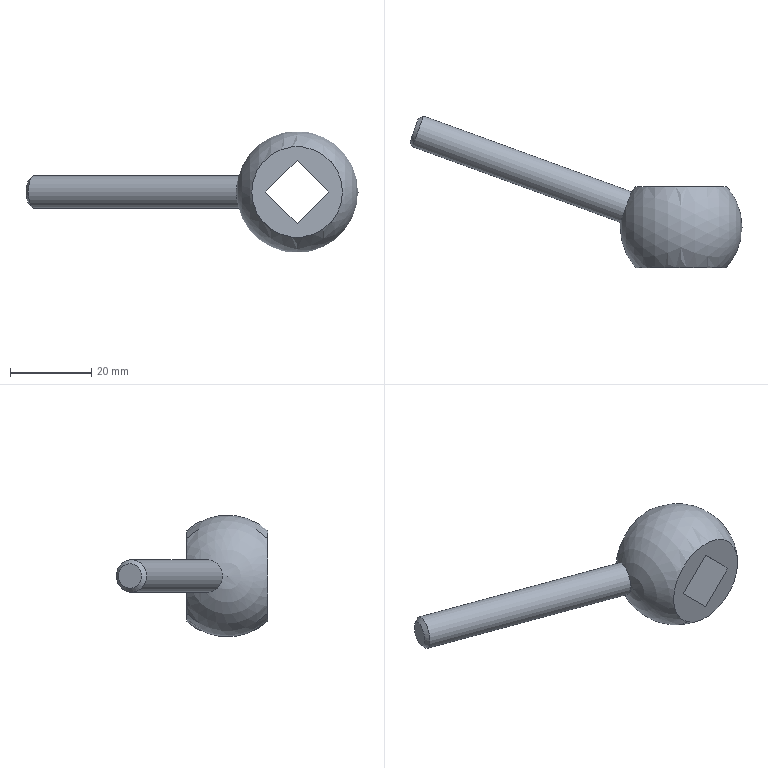Component | NX | HANDLE | 1 solid | 10 faces | box 81.8 x 37.36 x 30 mm | volume 12389 mm3 | plane 7 | sphere 1 | cylinder 1 | cone 1 | commonest cylinder face diameters 8 x1
STEP:
#1=CARTESIAN_POINT('',(0.,0.,0.));
#2=DIRECTION('',(0.,0.,1.));
#3=DIRECTION('',(1.,0.,0.));
#4=AXIS2_PLACEMENT_3D('',#1,#2,#3);
#5=CARTESIAN_POINT('',(11.18,65.,66.));
#6=VERTEX_POINT('',#5);
#7=CARTESIAN_POINT('',(0.,65.,66.));
#8=DIRECTION('',(0.,-1.,0.));
#9=DIRECTION('',(1.,0.,0.));
#10=AXIS2_PLACEMENT_3D('',#7,#8,#9);
#11=CIRCLE('',#10,11.18);
#12=CARTESIAN_POINT('',(0.,65.,66.));
#13=DIRECTION('',(0.,1.,0.));
#14=DIRECTION('',(1.,0.,0.));
#15=AXIS2_PLACEMENT_3D('',#12,#13,#14);
#16=PLANE('',#15);
#17=CARTESIAN_POINT('',(11.18,0.));
#18=CARTESIAN_POINT('',(11.18,-19.365));
#19=CARTESIAN_POINT('',(-5.59,-9.682));
#20=CARTESIAN_POINT('',(-22.361,-0.));
#21=CARTESIAN_POINT('',(-5.59,9.682));
#22=CARTESIAN_POINT('',(11.18,19.365));
#23=CARTESIAN_POINT('',(11.18,0.));
#24=(BOUNDED_CURVE()B_SPLINE_CURVE(2,(#17,#18,#19,#20,#21,#22,#23),.UNSPECIFIED.,.T.,.F.)B_SPLINE_CURVE_WITH_KNOTS((1,2,2,2,2,1),(-2.094,0.,2.094,4.189,6.283,8.378),.UNSPECIFIED.)CURVE()GEOMETRIC_REPRESENTATION_ITEM()RATIONAL_B_SPLINE_CURVE((1.,0.5,1.,0.5,1.,0.5,1.))REPRESENTATION_ITEM(''));
#25=(GEOMETRIC_REPRESENTATION_CONTEXT(2)PARAMETRIC_REPRESENTATION_CONTEXT()REPRESENTATION_CONTEXT('',''));
#26=DEFINITIONAL_REPRESENTATION('',(#24),#25);
#27=PCURVE('',#16,#26);
#28=CARTESIAN_POINT('',(0.,55.,66.));
#29=DIRECTION('',(-1.,0.,0.));
#30=DIRECTION('',(0.,1.,0.));
#31=AXIS2_PLACEMENT_3D('',#28,#29,#30);
#32=SPHERICAL_SURFACE('',#31,15.);
#33=CARTESIAN_POINT('',(6.283,-0.8411));
#34=CARTESIAN_POINT('',(6.172,-0.8417));
#35=CARTESIAN_POINT('',(5.967,-0.8094));
#36=CARTESIAN_POINT('',(5.725,-0.6857));
#37=CARTESIAN_POINT('',(5.571,-0.5142));
#38=CARTESIAN_POINT('',(5.481,-0.3169));
#39=CARTESIAN_POINT('',(5.44,-0.1069));
#40=CARTESIAN_POINT('',(5.44,0.1069));
#41=CARTESIAN_POINT('',(5.481,0.3169));
#42=CARTESIAN_POINT('',(5.571,0.5142));
#43=CARTESIAN_POINT('',(5.725,0.6856));
#44=CARTESIAN_POINT('',(5.965,0.8097));
#45=CARTESIAN_POINT('',(6.283,0.8568));
#46=CARTESIAN_POINT('',(6.601,0.8097));
#47=CARTESIAN_POINT('',(6.841,0.6856));
#48=CARTESIAN_POINT('',(6.996,0.5142));
#49=CARTESIAN_POINT('',(7.085,0.3169));
#50=CARTESIAN_POINT('',(7.126,0.1069));
#51=CARTESIAN_POINT('',(7.126,-0.1069));
#52=CARTESIAN_POINT('',(7.085,-0.3169));
#53=CARTESIAN_POINT('',(6.995,-0.5142));
#54=CARTESIAN_POINT('',(6.842,-0.6857));
#55=CARTESIAN_POINT('',(6.599,-0.8094));
#56=CARTESIAN_POINT('',(6.394,-0.8417));
#57=CARTESIAN_POINT('',(6.283,-0.8411));
#58=B_SPLINE_CURVE_WITH_KNOTS('',3,(#33,#34,#35,#36,#37,#38,#39,#40,#41,#42,#43,#44,#45,#46,#47,#48,#49,#50,#51,#52,#53,#54,#55,#56,#57),.UNSPECIFIED.,.T.,.F.,(4,1,1,1,1,1,1,1,1,1,1,1,1,1,1,1,1,1,1,1,1,1,4),(0.,0.2856,0.5712,0.8568,1.142,1.428,1.714,1.999,2.285,2.57,2.856,3.142,3.427,3.713,3.998,4.284,4.57,4.855,5.141,5.426,5.712,5.998,6.283),.QUASI_UNIFORM_KNOTS.);
#59=(GEOMETRIC_REPRESENTATION_CONTEXT(2)PARAMETRIC_REPRESENTATION_CONTEXT()REPRESENTATION_CONTEXT('',''));
#60=DEFINITIONAL_REPRESENTATION('',(#58),#59);
#61=PCURVE('',#32,#60);
#62=SURFACE_CURVE('',#11,(#27,#61),.PCURVE_S1.);
#63=EDGE_CURVE('',#6,#6,#62,.T.);
#64=ORIENTED_EDGE('',*,*,#63,.F.);
#65=EDGE_LOOP('',(#64));
#66=FACE_BOUND('',#65,.T.);
#67=CARTESIAN_POINT('',(0.,65.,58.222));
#68=VERTEX_POINT('',#67);
#69=CARTESIAN_POINT('',(7.778,65.,66.));
#70=VERTEX_POINT('',#69);
#71=CARTESIAN_POINT('',(3.889,65.,62.111));
#72=DIRECTION('',(0.7071,0.,0.7071));
#73=VECTOR('',#72,1.);
#74=LINE('',#71,#73);
#75=CARTESIAN_POINT('',(3.889,3.889));
#76=DIRECTION('',(0.7071,-0.7071));
#77=VECTOR('',#76,1.);
#78=LINE('',#75,#77);
#79=(GEOMETRIC_REPRESENTATION_CONTEXT(2)PARAMETRIC_REPRESENTATION_CONTEXT()REPRESENTATION_CONTEXT('',''));
#80=DEFINITIONAL_REPRESENTATION('',(#78),#79);
#81=PCURVE('',#16,#80);
#82=CARTESIAN_POINT('',(7.778,86.,66.));
#83=DIRECTION('',(-0.7071,0.,0.7071));
#84=DIRECTION('',(0.7071,0.,0.7071));
#85=AXIS2_PLACEMENT_3D('',#82,#83,#84);
#86=PLANE('',#85);
#87=CARTESIAN_POINT('',(-5.5,-21.));
#88=DIRECTION('',(1.,0.));
#89=VECTOR('',#88,1.);
#90=LINE('',#87,#89);
#91=(GEOMETRIC_REPRESENTATION_CONTEXT(2)PARAMETRIC_REPRESENTATION_CONTEXT()REPRESENTATION_CONTEXT('',''));
#92=DEFINITIONAL_REPRESENTATION('',(#90),#91);
#93=PCURVE('',#86,#92);
#94=SURFACE_CURVE('',#74,(#81,#93),.PCURVE_S1.);
#95=EDGE_CURVE('',#68,#70,#94,.T.);
#96=ORIENTED_EDGE('',*,*,#95,.T.);
#97=CARTESIAN_POINT('',(0.,65.,73.778));
#98=VERTEX_POINT('',#97);
#99=CARTESIAN_POINT('',(3.889,65.,69.889));
#100=DIRECTION('',(-0.7071,0.,0.7071));
#101=VECTOR('',#100,1.);
#102=LINE('',#99,#101);
#103=CARTESIAN_POINT('',(3.889,-3.889));
#104=DIRECTION('',(-0.7071,-0.7071));
#105=VECTOR('',#104,1.);
#106=LINE('',#103,#105);
#107=(GEOMETRIC_REPRESENTATION_CONTEXT(2)PARAMETRIC_REPRESENTATION_CONTEXT()REPRESENTATION_CONTEXT('',''));
#108=DEFINITIONAL_REPRESENTATION('',(#106),#107);
#109=PCURVE('',#16,#108);
#110=CARTESIAN_POINT('',(0.,86.,73.778));
#111=DIRECTION('',(-0.7071,0.,-0.7071));
#112=DIRECTION('',(-0.7071,0.,0.7071));
#113=AXIS2_PLACEMENT_3D('',#110,#111,#112);
#114=PLANE('',#113);
#115=CARTESIAN_POINT('',(-5.5,-21.));
#116=DIRECTION('',(1.,0.));
#117=VECTOR('',#116,1.);
#118=LINE('',#115,#117);
#119=(GEOMETRIC_REPRESENTATION_CONTEXT(2)PARAMETRIC_REPRESENTATION_CONTEXT()REPRESENTATION_CONTEXT('',''));
#120=DEFINITIONAL_REPRESENTATION('',(#118),#119);
#121=PCURVE('',#114,#120);
#122=SURFACE_CURVE('',#102,(#109,#121),.PCURVE_S1.);
#123=EDGE_CURVE('',#70,#98,#122,.T.);
#124=ORIENTED_EDGE('',*,*,#123,.T.);
#125=CARTESIAN_POINT('',(-7.778,65.,66.));
#126=VERTEX_POINT('',#125);
#127=CARTESIAN_POINT('',(-3.889,65.,69.889));
#128=DIRECTION('',(-0.7071,0.,-0.7071));
#129=VECTOR('',#128,1.);
#130=LINE('',#127,#129);
#131=CARTESIAN_POINT('',(-3.889,-3.889));
#132=DIRECTION('',(-0.7071,0.7071));
#133=VECTOR('',#132,1.);
#134=LINE('',#131,#133);
#135=(GEOMETRIC_REPRESENTATION_CONTEXT(2)PARAMETRIC_REPRESENTATION_CONTEXT()REPRESENTATION_CONTEXT('',''));
#136=DEFINITIONAL_REPRESENTATION('',(#134),#135);
#137=PCURVE('',#16,#136);
#138=CARTESIAN_POINT('',(-7.778,86.,66.));
#139=DIRECTION('',(0.7071,0.,-0.7071));
#140=DIRECTION('',(-0.7071,0.,-0.7071));
#141=AXIS2_PLACEMENT_3D('',#138,#139,#140);
#142=PLANE('',#141);
#143=CARTESIAN_POINT('',(-5.5,-21.));
#144=DIRECTION('',(1.,0.));
#145=VECTOR('',#144,1.);
#146=LINE('',#143,#145);
#147=(GEOMETRIC_REPRESENTATION_CONTEXT(2)PARAMETRIC_REPRESENTATION_CONTEXT()REPRESENTATION_CONTEXT('',''));
#148=DEFINITIONAL_REPRESENTATION('',(#146),#147);
#149=PCURVE('',#142,#148);
#150=SURFACE_CURVE('',#130,(#137,#149),.PCURVE_S1.);
#151=EDGE_CURVE('',#98,#126,#150,.T.);
#152=ORIENTED_EDGE('',*,*,#151,.T.);
#153=CARTESIAN_POINT('',(-3.889,65.,62.111));
#154=DIRECTION('',(0.7071,0.,-0.7071));
#155=VECTOR('',#154,1.);
#156=LINE('',#153,#155);
#157=CARTESIAN_POINT('',(-3.889,3.889));
#158=DIRECTION('',(0.7071,0.7071));
#159=VECTOR('',#158,1.);
#160=LINE('',#157,#159);
#161=(GEOMETRIC_REPRESENTATION_CONTEXT(2)PARAMETRIC_REPRESENTATION_CONTEXT()REPRESENTATION_CONTEXT('',''));
#162=DEFINITIONAL_REPRESENTATION('',(#160),#161);
#163=PCURVE('',#16,#162);
#164=CARTESIAN_POINT('',(0.,86.,58.222));
#165=DIRECTION('',(0.7071,0.,0.7071));
#166=DIRECTION('',(0.7071,0.,-0.7071));
#167=AXIS2_PLACEMENT_3D('',#164,#165,#166);
#168=PLANE('',#167);
#169=CARTESIAN_POINT('',(-5.5,-21.));
#170=DIRECTION('',(1.,0.));
#171=VECTOR('',#170,1.);
#172=LINE('',#169,#171);
#173=(GEOMETRIC_REPRESENTATION_CONTEXT(2)PARAMETRIC_REPRESENTATION_CONTEXT()REPRESENTATION_CONTEXT('',''));
#174=DEFINITIONAL_REPRESENTATION('',(#172),#173);
#175=PCURVE('',#168,#174);
#176=SURFACE_CURVE('',#156,(#163,#175),.PCURVE_S1.);
#177=EDGE_CURVE('',#126,#68,#176,.T.);
#178=ORIENTED_EDGE('',*,*,#177,.T.);
#179=EDGE_LOOP('',(#96,#124,#152,#178));
#180=FACE_BOUND('',#179,.T.);
#181=ADVANCED_FACE('',(#66,#180),#16,.T.);
#182=CARTESIAN_POINT('',(-11.18,45.,66.));
#183=VERTEX_POINT('',#182);
#184=CARTESIAN_POINT('',(0.,45.,66.));
#185=DIRECTION('',(0.,1.,0.));
#186=DIRECTION('',(-1.,0.,0.));
#187=AXIS2_PLACEMENT_3D('',#184,#185,#186);
#188=CIRCLE('',#187,11.18);
#189=CARTESIAN_POINT('',(0.,45.,66.));
#190=DIRECTION('',(0.,-1.,0.));
#191=DIRECTION('',(-1.,0.,0.));
#192=AXIS2_PLACEMENT_3D('',#189,#190,#191);
#193=PLANE('',#192);
#194=CARTESIAN_POINT('',(11.18,0.));
#195=CARTESIAN_POINT('',(11.18,-19.365));
#196=CARTESIAN_POINT('',(-5.59,-9.682));
#197=CARTESIAN_POINT('',(-22.361,-0.));
#198=CARTESIAN_POINT('',(-5.59,9.682));
#199=CARTESIAN_POINT('',(11.18,19.365));
#200=CARTESIAN_POINT('',(11.18,0.));
#201=(BOUNDED_CURVE()B_SPLINE_CURVE(2,(#194,#195,#196,#197,#198,#199,#200),.UNSPECIFIED.,.T.,.F.)B_SPLINE_CURVE_WITH_KNOTS((1,2,2,2,2,1),(-2.094,0.,2.094,4.189,6.283,8.378),.UNSPECIFIED.)CURVE()GEOMETRIC_REPRESENTATION_ITEM()RATIONAL_B_SPLINE_CURVE((1.,0.5,1.,0.5,1.,0.5,1.))REPRESENTATION_ITEM(''));
#202=(GEOMETRIC_REPRESENTATION_CONTEXT(2)PARAMETRIC_REPRESENTATION_CONTEXT()REPRESENTATION_CONTEXT('',''));
#203=DEFINITIONAL_REPRESENTATION('',(#201),#202);
#204=PCURVE('',#193,#203);
#205=CARTESIAN_POINT('',(9.425,0.8411));
#206=CARTESIAN_POINT('',(9.536,0.8417));
#207=CARTESIAN_POINT('',(9.741,0.8094));
#208=CARTESIAN_POINT('',(9.983,0.6857));
#209=CARTESIAN_POINT('',(10.137,0.5142));
#210=CARTESIAN_POINT('',(10.227,0.3169));
#211=CARTESIAN_POINT('',(10.268,0.1069));
#212=CARTESIAN_POINT('',(10.268,-0.1069));
#213=CARTESIAN_POINT('',(10.227,-0.3169));
#214=CARTESIAN_POINT('',(10.137,-0.5142));
#215=CARTESIAN_POINT('',(9.983,-0.6856));
#216=CARTESIAN_POINT('',(9.743,-0.8097));
#217=CARTESIAN_POINT('',(9.425,-0.8568));
#218=CARTESIAN_POINT('',(9.107,-0.8097));
#219=CARTESIAN_POINT('',(8.867,-0.6856));
#220=CARTESIAN_POINT('',(8.712,-0.5142));
#221=CARTESIAN_POINT('',(8.623,-0.3169));
#222=CARTESIAN_POINT('',(8.582,-0.1069));
#223=CARTESIAN_POINT('',(8.582,0.1069));
#224=CARTESIAN_POINT('',(8.623,0.3169));
#225=CARTESIAN_POINT('',(8.713,0.5142));
#226=CARTESIAN_POINT('',(8.866,0.6857));
#227=CARTESIAN_POINT('',(9.109,0.8094));
#228=CARTESIAN_POINT('',(9.314,0.8417));
#229=CARTESIAN_POINT('',(9.425,0.8411));
#230=B_SPLINE_CURVE_WITH_KNOTS('',3,(#205,#206,#207,#208,#209,#210,#211,#212,#213,#214,#215,#216,#217,#218,#219,#220,#221,#222,#223,#224,#225,#226,#227,#228,#229),.UNSPECIFIED.,.T.,.F.,(4,1,1,1,1,1,1,1,1,1,1,1,1,1,1,1,1,1,1,1,1,1,4),(0.,0.2856,0.5712,0.8568,1.142,1.428,1.714,1.999,2.285,2.57,2.856,3.142,3.427,3.713,3.998,4.284,4.57,4.855,5.141,5.426,5.712,5.998,6.283),.QUASI_UNIFORM_KNOTS.);
#231=(GEOMETRIC_REPRESENTATION_CONTEXT(2)PARAMETRIC_REPRESENTATION_CONTEXT()REPRESENTATION_CONTEXT('',''));
#232=DEFINITIONAL_REPRESENTATION('',(#230),#231);
#233=PCURVE('',#32,#232);
#234=SURFACE_CURVE('',#188,(#204,#233),.PCURVE_S1.);
#235=EDGE_CURVE('',#183,#183,#234,.T.);
#236=ORIENTED_EDGE('',*,*,#235,.F.);
#237=EDGE_LOOP('',(#236));
#238=FACE_BOUND('',#237,.T.);
#239=CARTESIAN_POINT('',(-7.778,45.,66.));
#240=VERTEX_POINT('',#239);
#241=CARTESIAN_POINT('',(0.,45.,73.778));
#242=VERTEX_POINT('',#241);
#243=CARTESIAN_POINT('',(-3.889,45.,69.889));
#244=DIRECTION('',(0.7071,0.,0.7071));
#245=VECTOR('',#244,1.);
#246=LINE('',#243,#245);
#247=CARTESIAN_POINT('',(3.889,-3.889));
#248=DIRECTION('',(-0.7071,-0.7071));
#249=VECTOR('',#248,1.);
#250=LINE('',#247,#249);
#251=(GEOMETRIC_REPRESENTATION_CONTEXT(2)PARAMETRIC_REPRESENTATION_CONTEXT()REPRESENTATION_CONTEXT('',''));
#252=DEFINITIONAL_REPRESENTATION('',(#250),#251);
#253=PCURVE('',#193,#252);
#254=CARTESIAN_POINT('',(-5.5,-41.));
#255=DIRECTION('',(-1.,0.));
#256=VECTOR('',#255,1.);
#257=LINE('',#254,#256);
#258=(GEOMETRIC_REPRESENTATION_CONTEXT(2)PARAMETRIC_REPRESENTATION_CONTEXT()REPRESENTATION_CONTEXT('',''));
#259=DEFINITIONAL_REPRESENTATION('',(#257),#258);
#260=PCURVE('',#142,#259);
#261=SURFACE_CURVE('',#246,(#253,#260),.PCURVE_S1.);
#262=EDGE_CURVE('',#240,#242,#261,.T.);
#263=ORIENTED_EDGE('',*,*,#262,.T.);
#264=CARTESIAN_POINT('',(7.778,45.,66.));
#265=VERTEX_POINT('',#264);
#266=CARTESIAN_POINT('',(3.889,45.,69.889));
#267=DIRECTION('',(0.7071,0.,-0.7071));
#268=VECTOR('',#267,1.);
#269=LINE('',#266,#268);
#270=CARTESIAN_POINT('',(-3.889,-3.889));
#271=DIRECTION('',(-0.7071,0.7071));
#272=VECTOR('',#271,1.);
#273=LINE('',#270,#272);
#274=(GEOMETRIC_REPRESENTATION_CONTEXT(2)PARAMETRIC_REPRESENTATION_CONTEXT()REPRESENTATION_CONTEXT('',''));
#275=DEFINITIONAL_REPRESENTATION('',(#273),#274);
#276=PCURVE('',#193,#275);
#277=CARTESIAN_POINT('',(-5.5,-41.));
#278=DIRECTION('',(-1.,0.));
#279=VECTOR('',#278,1.);
#280=LINE('',#277,#279);
#281=(GEOMETRIC_REPRESENTATION_CONTEXT(2)PARAMETRIC_REPRESENTATION_CONTEXT()REPRESENTATION_CONTEXT('',''));
#282=DEFINITIONAL_REPRESENTATION('',(#280),#281);
#283=PCURVE('',#114,#282);
#284=SURFACE_CURVE('',#269,(#276,#283),.PCURVE_S1.);
#285=EDGE_CURVE('',#242,#265,#284,.T.);
#286=ORIENTED_EDGE('',*,*,#285,.T.);
#287=CARTESIAN_POINT('',(0.,45.,58.222));
#288=VERTEX_POINT('',#287);
#289=CARTESIAN_POINT('',(3.889,45.,62.111));
#290=DIRECTION('',(-0.7071,0.,-0.7071));
#291=VECTOR('',#290,1.);
#292=LINE('',#289,#291);
#293=CARTESIAN_POINT('',(-3.889,3.889));
#294=DIRECTION('',(0.7071,0.7071));
#295=VECTOR('',#294,1.);
#296=LINE('',#293,#295);
#297=(GEOMETRIC_REPRESENTATION_CONTEXT(2)PARAMETRIC_REPRESENTATION_CONTEXT()REPRESENTATION_CONTEXT('',''));
#298=DEFINITIONAL_REPRESENTATION('',(#296),#297);
#299=PCURVE('',#193,#298);
#300=CARTESIAN_POINT('',(-5.5,-41.));
#301=DIRECTION('',(-1.,0.));
#302=VECTOR('',#301,1.);
#303=LINE('',#300,#302);
#304=(GEOMETRIC_REPRESENTATION_CONTEXT(2)PARAMETRIC_REPRESENTATION_CONTEXT()REPRESENTATION_CONTEXT('',''));
#305=DEFINITIONAL_REPRESENTATION('',(#303),#304);
#306=PCURVE('',#86,#305);
#307=SURFACE_CURVE('',#292,(#299,#306),.PCURVE_S1.);
#308=EDGE_CURVE('',#265,#288,#307,.T.);
#309=ORIENTED_EDGE('',*,*,#308,.T.);
#310=CARTESIAN_POINT('',(-3.889,45.,62.111));
#311=DIRECTION('',(-0.7071,0.,0.7071));
#312=VECTOR('',#311,1.);
#313=LINE('',#310,#312);
#314=CARTESIAN_POINT('',(3.889,3.889));
#315=DIRECTION('',(0.7071,-0.7071));
#316=VECTOR('',#315,1.);
#317=LINE('',#314,#316);
#318=(GEOMETRIC_REPRESENTATION_CONTEXT(2)PARAMETRIC_REPRESENTATION_CONTEXT()REPRESENTATION_CONTEXT('',''));
#319=DEFINITIONAL_REPRESENTATION('',(#317),#318);
#320=PCURVE('',#193,#319);
#321=CARTESIAN_POINT('',(-5.5,-41.));
#322=DIRECTION('',(-1.,0.));
#323=VECTOR('',#322,1.);
#324=LINE('',#321,#323);
#325=(GEOMETRIC_REPRESENTATION_CONTEXT(2)PARAMETRIC_REPRESENTATION_CONTEXT()REPRESENTATION_CONTEXT('',''));
#326=DEFINITIONAL_REPRESENTATION('',(#324),#325);
#327=PCURVE('',#168,#326);
#328=SURFACE_CURVE('',#313,(#320,#327),.PCURVE_S1.);
#329=EDGE_CURVE('',#288,#240,#328,.T.);
#330=ORIENTED_EDGE('',*,*,#329,.T.);
#331=EDGE_LOOP('',(#263,#286,#309,#330));
#332=FACE_BOUND('',#331,.T.);
#333=ADVANCED_FACE('',(#238,#332),#193,.T.);
#334=ORIENTED_EDGE('',*,*,#235,.T.);
#335=EDGE_LOOP('',(#334));
#336=FACE_BOUND('',#335,.T.);
#337=ORIENTED_EDGE('',*,*,#63,.T.);
#338=EDGE_LOOP('',(#337));
#339=FACE_BOUND('',#338,.T.);
#340=CARTESIAN_POINT('',(-14.953,56.186,66.));
#341=VERTEX_POINT('',#340);
#342=CARTESIAN_POINT('',(-13.585,59.945,66.));
#343=DIRECTION('',(0.9397,-0.342,0.));
#344=DIRECTION('',(-0.342,-0.9397,0.));
#345=AXIS2_PLACEMENT_3D('',#342,#343,#344);
#346=CIRCLE('',#345,4.);
#347=CARTESIAN_POINT('',(6.283,1.492));
#348=CARTESIAN_POINT('',(6.641,1.488));
#349=CARTESIAN_POINT('',(7.072,1.46));
#350=CARTESIAN_POINT('',(7.185,1.383));
#351=CARTESIAN_POINT('',(7.176,1.307));
#352=CARTESIAN_POINT('',(7.109,1.232));
#353=CARTESIAN_POINT('',(7.017,1.163));
#354=CARTESIAN_POINT('',(6.91,1.102));
#355=CARTESIAN_POINT('',(6.794,1.049));
#356=CARTESIAN_POINT('',(6.671,1.006));
#357=CARTESIAN_POINT('',(6.544,0.9752));
#358=CARTESIAN_POINT('',(6.414,0.9561));
#359=CARTESIAN_POINT('',(6.283,0.9497));
#360=CARTESIAN_POINT('',(6.152,0.9561));
#361=CARTESIAN_POINT('',(6.022,0.9752));
#362=CARTESIAN_POINT('',(5.895,1.006));
#363=CARTESIAN_POINT('',(5.772,1.049));
#364=CARTESIAN_POINT('',(5.656,1.102));
#365=CARTESIAN_POINT('',(5.549,1.163));
#366=CARTESIAN_POINT('',(5.457,1.232));
#367=CARTESIAN_POINT('',(5.39,1.307));
#368=CARTESIAN_POINT('',(5.382,1.383));
#369=CARTESIAN_POINT('',(5.494,1.46));
#370=CARTESIAN_POINT('',(5.926,1.488));
#371=CARTESIAN_POINT('',(6.283,1.492));
#372=B_SPLINE_CURVE_WITH_KNOTS('',3,(#347,#348,#349,#350,#351,#352,#353,#354,#355,#356,#357,#358,#359,#360,#361,#362,#363,#364,#365,#366,#367,#368,#369,#370,#371),.UNSPECIFIED.,.T.,.F.,(4,1,1,1,1,1,1,1,1,1,1,1,1,1,1,1,1,1,1,1,1,1,4),(0.,0.2856,0.5712,0.8568,1.142,1.428,1.714,1.999,2.285,2.57,2.856,3.142,3.427,3.713,3.998,4.284,4.57,4.855,5.141,5.426,5.712,5.998,6.283),.QUASI_UNIFORM_KNOTS.);
#373=(GEOMETRIC_REPRESENTATION_CONTEXT(2)PARAMETRIC_REPRESENTATION_CONTEXT()REPRESENTATION_CONTEXT('',''));
#374=DEFINITIONAL_REPRESENTATION('',(#372),#373);
#375=PCURVE('',#32,#374);
#376=CARTESIAN_POINT('',(0.,55.,66.));
#377=DIRECTION('',(-0.9397,0.342,0.));
#378=DIRECTION('',(0.342,0.9397,0.));
#379=AXIS2_PLACEMENT_3D('',#376,#377,#378);
#380=CYLINDRICAL_SURFACE('',#379,4.);
#381=CARTESIAN_POINT('',(9.425,14.457));
#382=DIRECTION('',(-1.,0.));
#383=VECTOR('',#382,1.);
#384=LINE('',#381,#383);
#385=(GEOMETRIC_REPRESENTATION_CONTEXT(2)PARAMETRIC_REPRESENTATION_CONTEXT()REPRESENTATION_CONTEXT('',''));
#386=DEFINITIONAL_REPRESENTATION('',(#384),#385);
#387=PCURVE('',#380,#386);
#388=SURFACE_CURVE('',#346,(#375,#387),.PCURVE_S1.);
#389=EDGE_CURVE('',#341,#341,#388,.T.);
#390=ORIENTED_EDGE('',*,*,#389,.T.);
#391=EDGE_LOOP('',(#390));
#392=FACE_BOUND('',#391,.T.);
#393=CARTESIAN_POINT('',(15.,55.,66.));
#394=VERTEX_POINT('',#393);
#395=VERTEX_LOOP('',#394);
#396=FACE_BOUND('',#395,.T.);
#397=ADVANCED_FACE('',(#336,#339,#392,#396),#32,.T.);
#398=CARTESIAN_POINT('',(-66.207,74.841,66.));
#399=VERTEX_POINT('',#398);
#400=CARTESIAN_POINT('',(-64.839,78.599,66.));
#401=DIRECTION('',(0.9397,-0.342,0.));
#402=DIRECTION('',(-0.342,-0.9397,0.));
#403=AXIS2_PLACEMENT_3D('',#400,#401,#402);
#404=CIRCLE('',#403,4.);
#405=CARTESIAN_POINT('',(9.425,69.));
#406=DIRECTION('',(-1.,0.));
#407=VECTOR('',#406,1.);
#408=LINE('',#405,#407);
#409=(GEOMETRIC_REPRESENTATION_CONTEXT(2)PARAMETRIC_REPRESENTATION_CONTEXT()REPRESENTATION_CONTEXT('',''));
#410=DEFINITIONAL_REPRESENTATION('',(#408),#409);
#411=PCURVE('',#380,#410);
#412=CARTESIAN_POINT('',(-64.839,78.599,66.));
#413=DIRECTION('',(0.9397,-0.342,0.));
#414=DIRECTION('',(-0.342,-0.9397,0.));
#415=AXIS2_PLACEMENT_3D('',#412,#413,#414);
#416=CONICAL_SURFACE('',#415,4.,0.7854);
#417=CARTESIAN_POINT('',(0.,0.));
#418=DIRECTION('',(1.,0.));
#419=VECTOR('',#418,1.);
#420=LINE('',#417,#419);
#421=(GEOMETRIC_REPRESENTATION_CONTEXT(2)PARAMETRIC_REPRESENTATION_CONTEXT()REPRESENTATION_CONTEXT('',''));
#422=DEFINITIONAL_REPRESENTATION('',(#420),#421);
#423=PCURVE('',#416,#422);
#424=SURFACE_CURVE('',#404,(#411,#423),.PCURVE_S1.);
#425=EDGE_CURVE('',#399,#399,#424,.T.);
#426=ORIENTED_EDGE('',*,*,#425,.T.);
#427=CARTESIAN_POINT('',(-14.953,56.186,66.));
#428=CARTESIAN_POINT('',(-66.207,74.841,66.));
#429=B_SPLINE_CURVE_WITH_KNOTS('',1,(#427,#428),.UNSPECIFIED.,.F.,.F.,(2,2),(14.457,69.),.PIECEWISE_BEZIER_KNOTS.);
#430=CARTESIAN_POINT('',(3.142,0.));
#431=DIRECTION('',(0.,1.));
#432=VECTOR('',#431,1.);
#433=LINE('',#430,#432);
#434=(GEOMETRIC_REPRESENTATION_CONTEXT(2)PARAMETRIC_REPRESENTATION_CONTEXT()REPRESENTATION_CONTEXT('',''));
#435=DEFINITIONAL_REPRESENTATION('',(#433),#434);
#436=PCURVE('',#380,#435);
#437=CARTESIAN_POINT('',(9.425,0.));
#438=DIRECTION('',(0.,1.));
#439=VECTOR('',#438,1.);
#440=LINE('',#437,#439);
#441=(GEOMETRIC_REPRESENTATION_CONTEXT(2)PARAMETRIC_REPRESENTATION_CONTEXT()REPRESENTATION_CONTEXT('',''));
#442=DEFINITIONAL_REPRESENTATION('',(#440),#441);
#443=PCURVE('',#380,#442);
#444=SEAM_CURVE('',#429,(#436,#443),.PCURVE_S1.);
#445=EDGE_CURVE('',#341,#399,#444,.T.);
#446=ORIENTED_EDGE('',*,*,#445,.F.);
#447=ORIENTED_EDGE('',*,*,#389,.F.);
#448=ORIENTED_EDGE('',*,*,#445,.T.);
#449=EDGE_LOOP('',(#426,#446,#447,#448));
#450=FACE_BOUND('',#449,.T.);
#451=ADVANCED_FACE('',(#450),#380,.T.);
#452=CARTESIAN_POINT('',(-66.805,76.122,66.));
#453=VERTEX_POINT('',#452);
#454=CARTESIAN_POINT('',(-65.778,78.941,66.));
#455=DIRECTION('',(-0.9397,0.342,0.));
#456=DIRECTION('',(-0.342,-0.9397,0.));
#457=AXIS2_PLACEMENT_3D('',#454,#455,#456);
#458=CIRCLE('',#457,3.);
#459=CARTESIAN_POINT('',(-65.778,78.941,66.));
#460=DIRECTION('',(0.9397,-0.342,0.));
#461=DIRECTION('',(-0.342,-0.9397,0.));
#462=AXIS2_PLACEMENT_3D('',#459,#460,#461);
#463=PLANE('',#462);
#464=CARTESIAN_POINT('',(3.,0.));
#465=CARTESIAN_POINT('',(3.,-5.196));
#466=CARTESIAN_POINT('',(-1.5,-2.598));
#467=CARTESIAN_POINT('',(-6.,-0.));
#468=CARTESIAN_POINT('',(-1.5,2.598));
#469=CARTESIAN_POINT('',(3.,5.196));
#470=CARTESIAN_POINT('',(3.,0.));
#471=(BOUNDED_CURVE()B_SPLINE_CURVE(2,(#464,#465,#466,#467,#468,#469,#470),.UNSPECIFIED.,.T.,.F.)B_SPLINE_CURVE_WITH_KNOTS((1,2,2,2,2,1),(-2.094,0.,2.094,4.189,6.283,8.378),.UNSPECIFIED.)CURVE()GEOMETRIC_REPRESENTATION_ITEM()RATIONAL_B_SPLINE_CURVE((1.,0.5,1.,0.5,1.,0.5,1.))REPRESENTATION_ITEM(''));
#472=(GEOMETRIC_REPRESENTATION_CONTEXT(2)PARAMETRIC_REPRESENTATION_CONTEXT()REPRESENTATION_CONTEXT('',''));
#473=DEFINITIONAL_REPRESENTATION('',(#471),#472);
#474=PCURVE('',#463,#473);
#475=CARTESIAN_POINT('',(6.283,-1.));
#476=DIRECTION('',(-1.,0.));
#477=VECTOR('',#476,1.);
#478=LINE('',#475,#477);
#479=(GEOMETRIC_REPRESENTATION_CONTEXT(2)PARAMETRIC_REPRESENTATION_CONTEXT()REPRESENTATION_CONTEXT('',''));
#480=DEFINITIONAL_REPRESENTATION('',(#478),#479);
#481=PCURVE('',#416,#480);
#482=SURFACE_CURVE('',#458,(#474,#481),.PCURVE_S1.);
#483=EDGE_CURVE('',#453,#453,#482,.T.);
#484=ORIENTED_EDGE('',*,*,#483,.T.);
#485=EDGE_LOOP('',(#484));
#486=FACE_BOUND('',#485,.T.);
#487=ADVANCED_FACE('',(#486),#463,.F.);
#488=CARTESIAN_POINT('',(7.778,86.,66.));
#489=DIRECTION('',(0.,1.,0.));
#490=VECTOR('',#489,1.);
#491=LINE('',#488,#490);
#492=CARTESIAN_POINT('',(-11.,0.));
#493=DIRECTION('',(0.,1.));
#494=VECTOR('',#493,1.);
#495=LINE('',#492,#494);
#496=(GEOMETRIC_REPRESENTATION_CONTEXT(2)PARAMETRIC_REPRESENTATION_CONTEXT()REPRESENTATION_CONTEXT('',''));
#497=DEFINITIONAL_REPRESENTATION('',(#495),#496);
#498=PCURVE('',#114,#497);
#499=CARTESIAN_POINT('',(0.,0.));
#500=DIRECTION('',(0.,1.));
#501=VECTOR('',#500,1.);
#502=LINE('',#499,#501);
#503=(GEOMETRIC_REPRESENTATION_CONTEXT(2)PARAMETRIC_REPRESENTATION_CONTEXT()REPRESENTATION_CONTEXT('',''));
#504=DEFINITIONAL_REPRESENTATION('',(#502),#503);
#505=PCURVE('',#86,#504);
#506=SURFACE_CURVE('',#491,(#498,#505),.PCURVE_S1.);
#507=EDGE_CURVE('',#265,#70,#506,.T.);
#508=ORIENTED_EDGE('',*,*,#507,.F.);
#509=ORIENTED_EDGE('',*,*,#285,.F.);
#510=CARTESIAN_POINT('',(0.,86.,73.778));
#511=DIRECTION('',(0.,1.,0.));
#512=VECTOR('',#511,1.);
#513=LINE('',#510,#512);
#514=CARTESIAN_POINT('',(0.,0.));
#515=DIRECTION('',(0.,1.));
#516=VECTOR('',#515,1.);
#517=LINE('',#514,#516);
#518=(GEOMETRIC_REPRESENTATION_CONTEXT(2)PARAMETRIC_REPRESENTATION_CONTEXT()REPRESENTATION_CONTEXT('',''));
#519=DEFINITIONAL_REPRESENTATION('',(#517),#518);
#520=PCURVE('',#114,#519);
#521=CARTESIAN_POINT('',(-11.,0.));
#522=DIRECTION('',(0.,1.));
#523=VECTOR('',#522,1.);
#524=LINE('',#521,#523);
#525=(GEOMETRIC_REPRESENTATION_CONTEXT(2)PARAMETRIC_REPRESENTATION_CONTEXT()REPRESENTATION_CONTEXT('',''));
#526=DEFINITIONAL_REPRESENTATION('',(#524),#525);
#527=PCURVE('',#142,#526);
#528=SURFACE_CURVE('',#513,(#520,#527),.PCURVE_S1.);
#529=EDGE_CURVE('',#242,#98,#528,.T.);
#530=ORIENTED_EDGE('',*,*,#529,.T.);
#531=ORIENTED_EDGE('',*,*,#123,.F.);
#532=EDGE_LOOP('',(#508,#509,#530,#531));
#533=FACE_BOUND('',#532,.T.);
#534=ADVANCED_FACE('',(#533),#114,.T.);
#535=CARTESIAN_POINT('',(0.,86.,58.222));
#536=DIRECTION('',(0.,1.,0.));
#537=VECTOR('',#536,1.);
#538=LINE('',#535,#537);
#539=CARTESIAN_POINT('',(-11.,0.));
#540=DIRECTION('',(0.,1.));
#541=VECTOR('',#540,1.);
#542=LINE('',#539,#541);
#543=(GEOMETRIC_REPRESENTATION_CONTEXT(2)PARAMETRIC_REPRESENTATION_CONTEXT()REPRESENTATION_CONTEXT('',''));
#544=DEFINITIONAL_REPRESENTATION('',(#542),#543);
#545=PCURVE('',#86,#544);
#546=CARTESIAN_POINT('',(0.,0.));
#547=DIRECTION('',(0.,1.));
#548=VECTOR('',#547,1.);
#549=LINE('',#546,#548);
#550=(GEOMETRIC_REPRESENTATION_CONTEXT(2)PARAMETRIC_REPRESENTATION_CONTEXT()REPRESENTATION_CONTEXT('',''));
#551=DEFINITIONAL_REPRESENTATION('',(#549),#550);
#552=PCURVE('',#168,#551);
#553=SURFACE_CURVE('',#538,(#545,#552),.PCURVE_S1.);
#554=EDGE_CURVE('',#288,#68,#553,.T.);
#555=ORIENTED_EDGE('',*,*,#554,.F.);
#556=ORIENTED_EDGE('',*,*,#308,.F.);
#557=ORIENTED_EDGE('',*,*,#507,.T.);
#558=ORIENTED_EDGE('',*,*,#95,.F.);
#559=EDGE_LOOP('',(#555,#556,#557,#558));
#560=FACE_BOUND('',#559,.T.);
#561=ADVANCED_FACE('',(#560),#86,.T.);
#562=CARTESIAN_POINT('',(-7.778,86.,66.));
#563=DIRECTION('',(0.,1.,0.));
#564=VECTOR('',#563,1.);
#565=LINE('',#562,#564);
#566=CARTESIAN_POINT('',(-11.,0.));
#567=DIRECTION('',(0.,1.));
#568=VECTOR('',#567,1.);
#569=LINE('',#566,#568);
#570=(GEOMETRIC_REPRESENTATION_CONTEXT(2)PARAMETRIC_REPRESENTATION_CONTEXT()REPRESENTATION_CONTEXT('',''));
#571=DEFINITIONAL_REPRESENTATION('',(#569),#570);
#572=PCURVE('',#168,#571);
#573=CARTESIAN_POINT('',(0.,0.));
#574=DIRECTION('',(0.,1.));
#575=VECTOR('',#574,1.);
#576=LINE('',#573,#575);
#577=(GEOMETRIC_REPRESENTATION_CONTEXT(2)PARAMETRIC_REPRESENTATION_CONTEXT()REPRESENTATION_CONTEXT('',''));
#578=DEFINITIONAL_REPRESENTATION('',(#576),#577);
#579=PCURVE('',#142,#578);
#580=SURFACE_CURVE('',#565,(#572,#579),.PCURVE_S1.);
#581=EDGE_CURVE('',#240,#126,#580,.T.);
#582=ORIENTED_EDGE('',*,*,#581,.F.);
#583=ORIENTED_EDGE('',*,*,#329,.F.);
#584=ORIENTED_EDGE('',*,*,#554,.T.);
#585=ORIENTED_EDGE('',*,*,#177,.F.);
#586=EDGE_LOOP('',(#582,#583,#584,#585));
#587=FACE_BOUND('',#586,.T.);
#588=ADVANCED_FACE('',(#587),#168,.T.);
#589=ORIENTED_EDGE('',*,*,#529,.F.);
#590=ORIENTED_EDGE('',*,*,#262,.F.);
#591=ORIENTED_EDGE('',*,*,#581,.T.);
#592=ORIENTED_EDGE('',*,*,#151,.F.);
#593=EDGE_LOOP('',(#589,#590,#591,#592));
#594=FACE_BOUND('',#593,.T.);
#595=ADVANCED_FACE('',(#594),#142,.T.);
#596=ORIENTED_EDGE('',*,*,#483,.F.);
#597=CARTESIAN_POINT('',(-66.805,76.122,66.));
#598=CARTESIAN_POINT('',(-66.207,74.841,66.));
#599=B_SPLINE_CURVE_WITH_KNOTS('',1,(#597,#598),.UNSPECIFIED.,.F.,.F.,(2,2),(-1.414,0.),.PIECEWISE_BEZIER_KNOTS.);
#600=CARTESIAN_POINT('',(6.283,0.));
#601=DIRECTION('',(0.,1.));
#602=VECTOR('',#601,1.);
#603=LINE('',#600,#602);
#604=(GEOMETRIC_REPRESENTATION_CONTEXT(2)PARAMETRIC_REPRESENTATION_CONTEXT()REPRESENTATION_CONTEXT('',''));
#605=DEFINITIONAL_REPRESENTATION('',(#603),#604);
#606=PCURVE('',#416,#605);
#607=CARTESIAN_POINT('',(0.,0.));
#608=DIRECTION('',(0.,1.));
#609=VECTOR('',#608,1.);
#610=LINE('',#607,#609);
#611=(GEOMETRIC_REPRESENTATION_CONTEXT(2)PARAMETRIC_REPRESENTATION_CONTEXT()REPRESENTATION_CONTEXT('',''));
#612=DEFINITIONAL_REPRESENTATION('',(#610),#611);
#613=PCURVE('',#416,#612);
#614=SEAM_CURVE('',#599,(#606,#613),.PCURVE_S1.);
#615=EDGE_CURVE('',#453,#399,#614,.T.);
#616=ORIENTED_EDGE('',*,*,#615,.T.);
#617=ORIENTED_EDGE('',*,*,#425,.F.);
#618=ORIENTED_EDGE('',*,*,#615,.F.);
#619=EDGE_LOOP('',(#596,#616,#617,#618));
#620=FACE_BOUND('',#619,.T.);
#621=ADVANCED_FACE('',(#620),#416,.T.);
#622=CLOSED_SHELL('',(#181,#333,#397,#451,#487,#534,#561,#588,#595,#621));
#623=MANIFOLD_SOLID_BREP('',#622);
#624=(LENGTH_UNIT()NAMED_UNIT(*)SI_UNIT(.MILLI.,.METRE.));
#625=UNCERTAINTY_MEASURE_WITH_UNIT(LENGTH_MEASURE(0.000002),#624,'','');
#626=(NAMED_UNIT(*)PLANE_ANGLE_UNIT()SI_UNIT($,.RADIAN.));
#627=(NAMED_UNIT(*)SI_UNIT($,.STERADIAN.)SOLID_ANGLE_UNIT());
#628=(GEOMETRIC_REPRESENTATION_CONTEXT(3)GLOBAL_UNCERTAINTY_ASSIGNED_CONTEXT((#625))GLOBAL_UNIT_ASSIGNED_CONTEXT((#624,#626,#627))REPRESENTATION_CONTEXT('',''));
#629=ADVANCED_BREP_SHAPE_REPRESENTATION('',(#4,#623),#628);